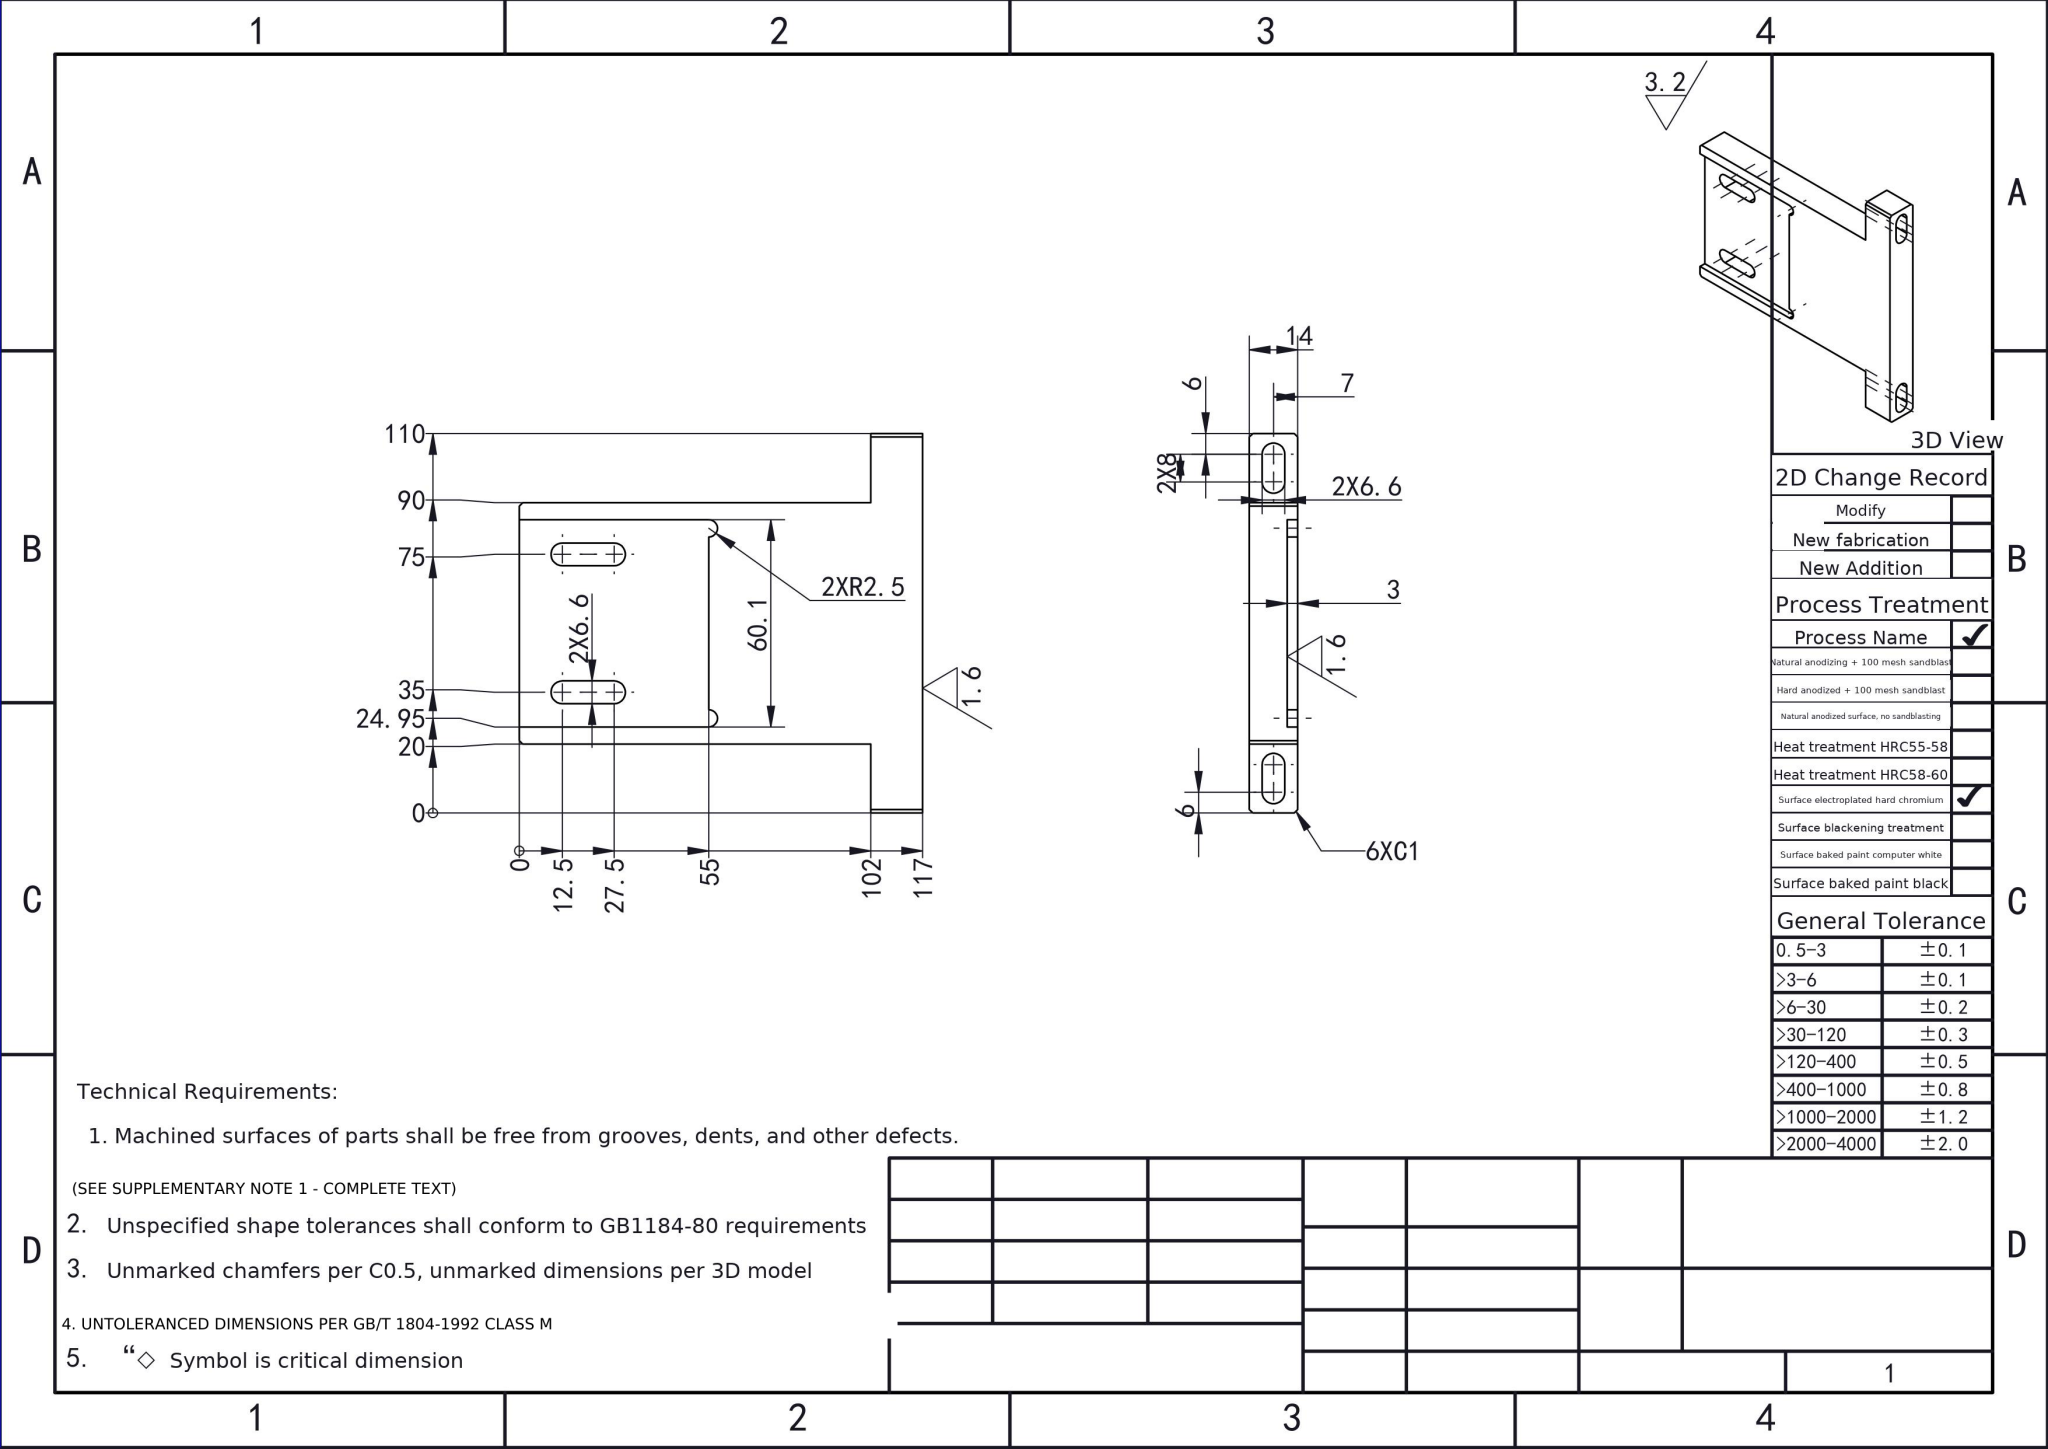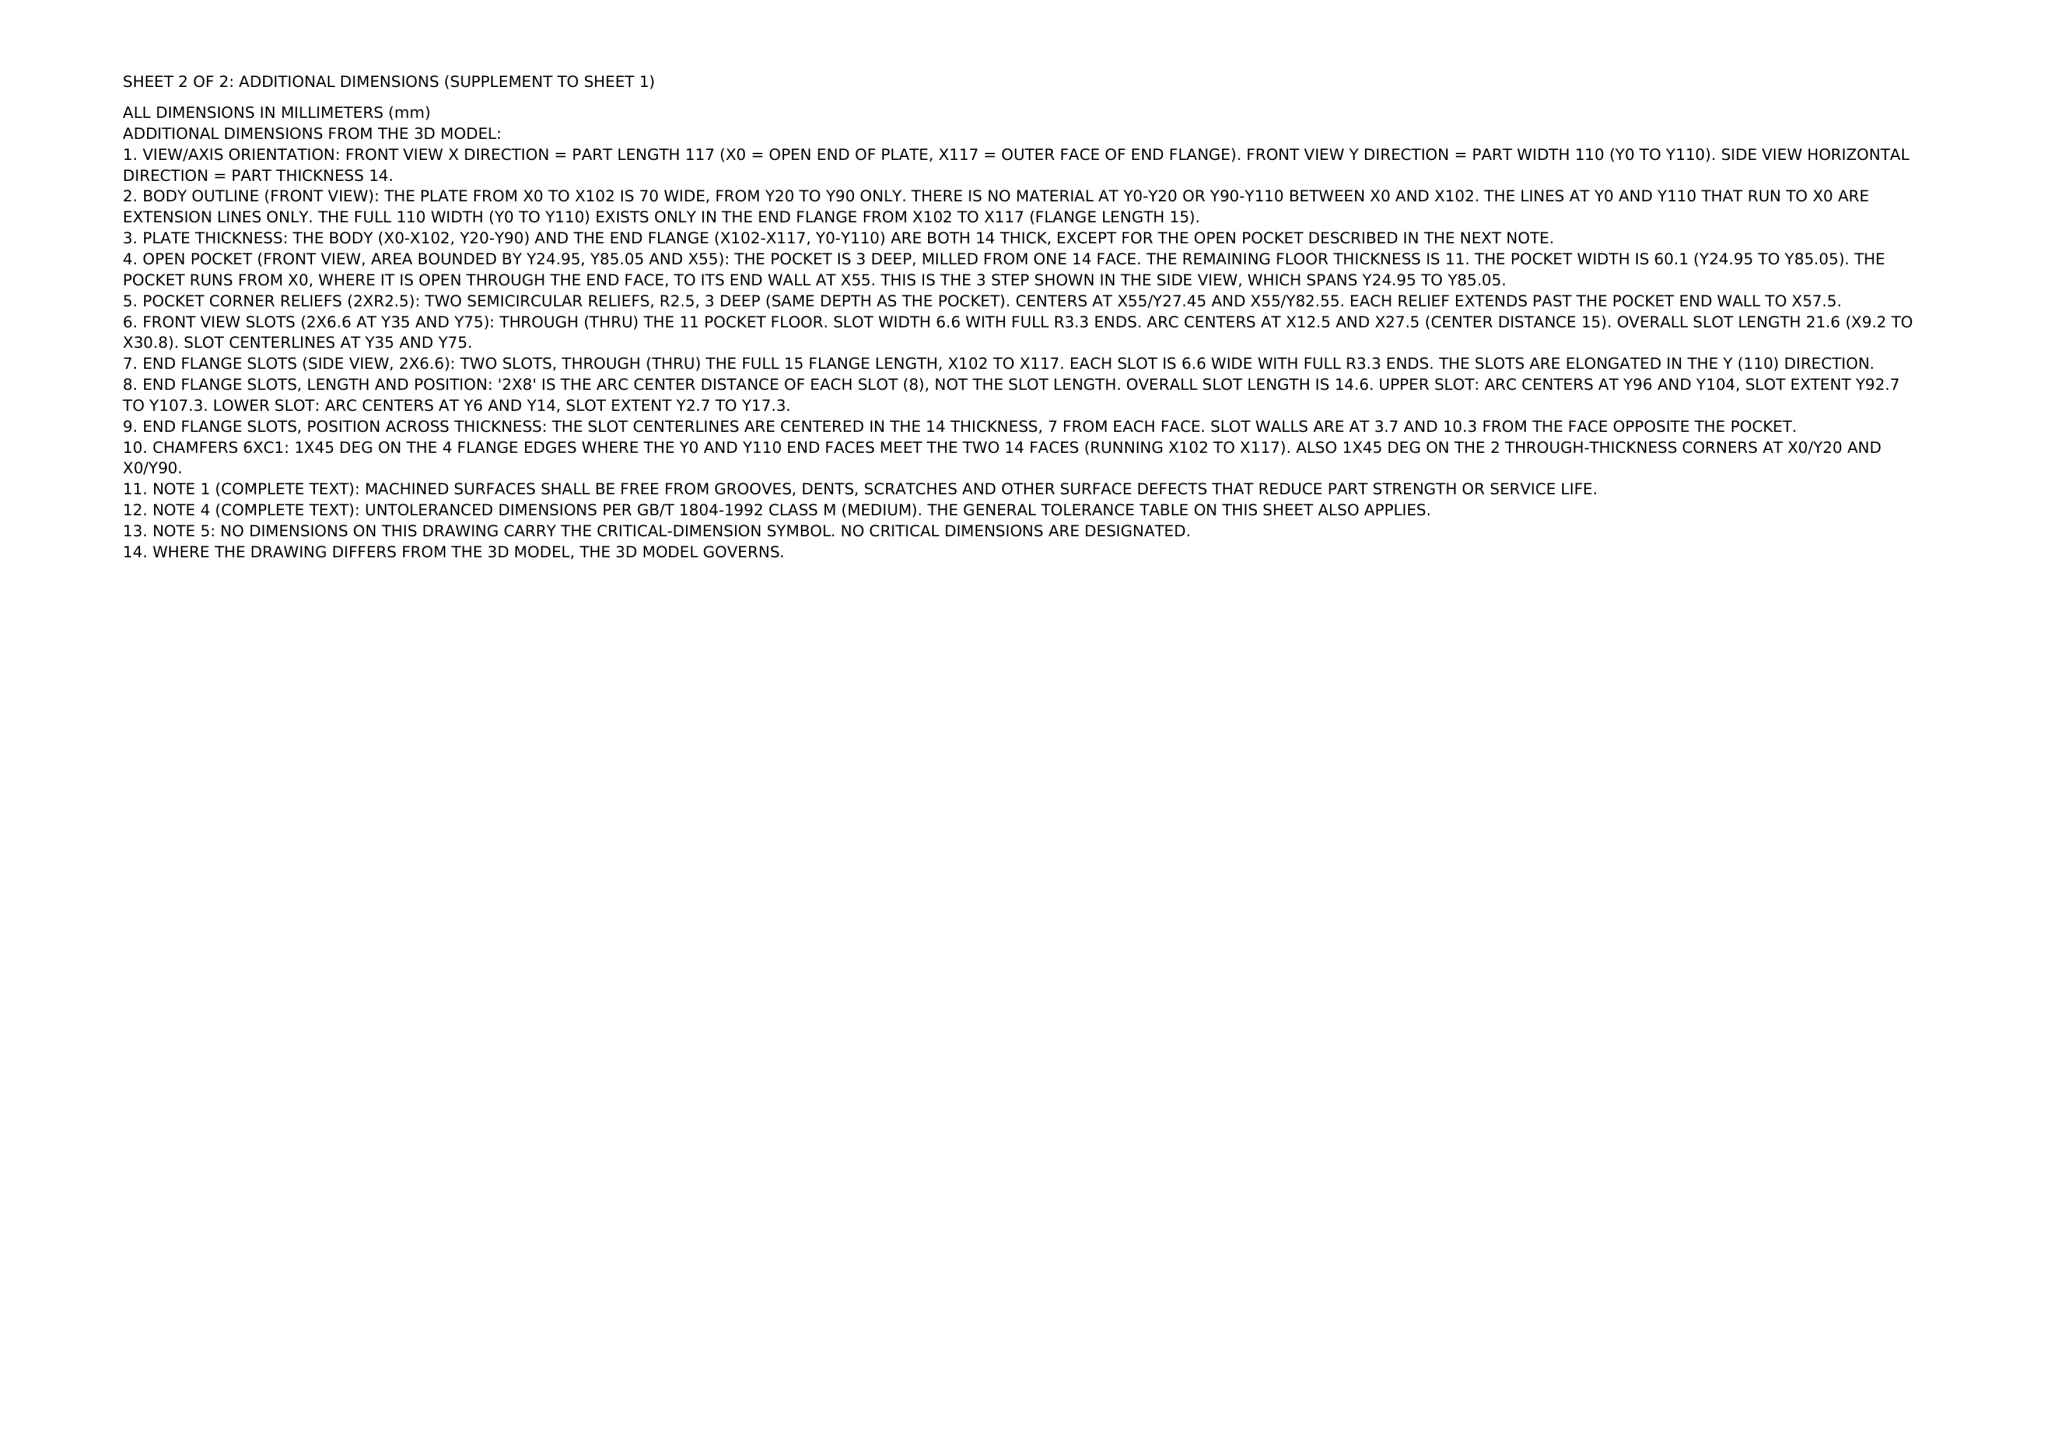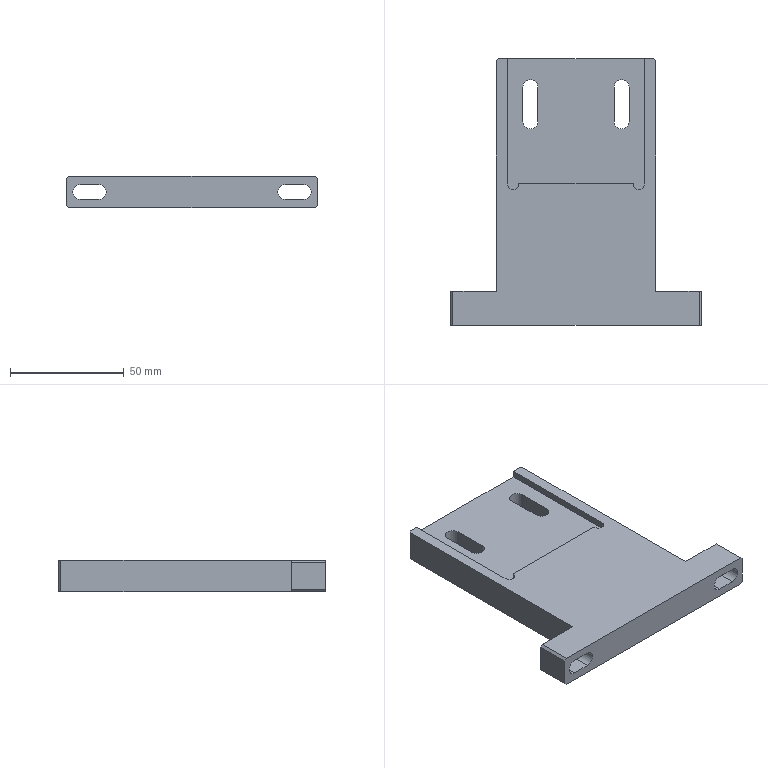Part | NX | mm | Stepped Slotted Mounting Tab | 1 solid | 38 faces | box 110 x 117 x 14 mm | volume 107500 mm3 | plane 28 | cylinder 10 | commonest cylinder face diameters 6.6 x8 5 x2